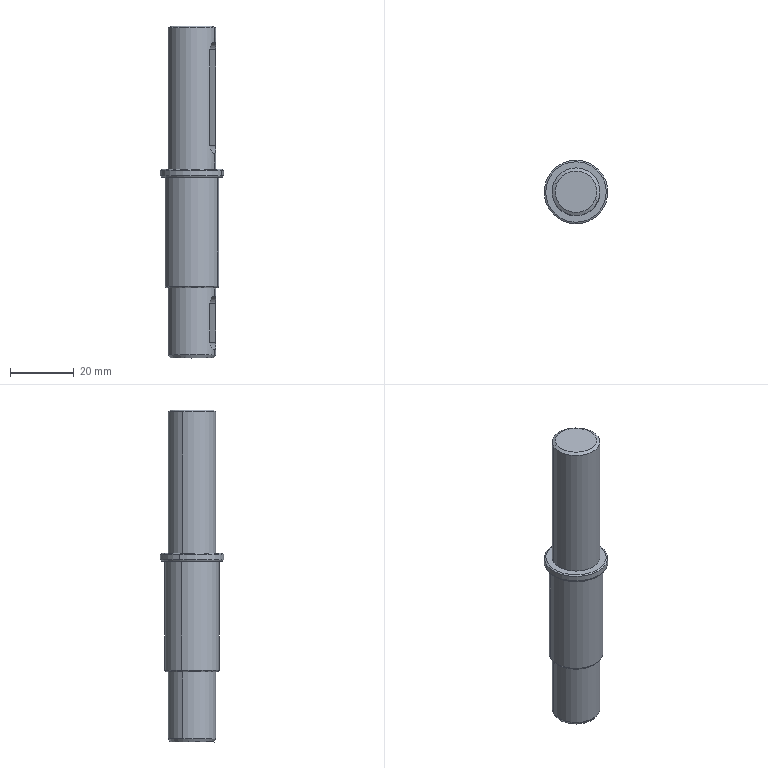Component | SolidWorks | 170423A4-ConveyorSynchronousPulleyAssembly-1_170423A4-PulleyFixedAxis1-1 | 1 solid | 35 faces | box 20 x 20 x 104.2 mm | volume 19748 mm3 | cylinder 14 | plane 11 | cone 10 | commonest cylinder face diameters 5 x6 15 x4 17 x2 20 x2
build123d program:
from build123d import *
from OCP.BRepFilletAPI import BRepFilletAPI_MakeChamfer

# Parameters (mm, degrees)
SKETCH1_R           = 7.5
BOSS_EXTRUDE1_DEPTH = 45
SKETCH2_R           = 10
BOSS_EXTRUDE2_DEPTH = 2.5
SKETCH3_R           = 8.5
BOSS_EXTRUDE3_DEPTH = 34.7
SKETCH4_R           = 7.5
BOSS_EXTRUDE4_DEPTH = 22
CHAMFER1_SIZE       = 1
CHAMFER1_SIZE2      = 0.5774
CHAMFER2_SIZE       = 0.5
CHAMFER2_SIZE2      = 0.2887
CUT_EXTRUDE3_DEPTH  = 3


with BuildPart() as part:
    # Sketch1 → Boss-Extrude1 (new body)
    with BuildSketch(Plane.XY):
        with Locations(Location((0, 0, 0), (0, 0, 180))):
            Circle(SKETCH1_R)
    extrude(amount=BOSS_EXTRUDE1_DEPTH)

    # Sketch2 → Boss-Extrude2 (add)
    with BuildSketch(Plane.XY.offset(45)):
        Circle(SKETCH2_R)
    extrude(amount=BOSS_EXTRUDE2_DEPTH)

    # Sketch3 → Boss-Extrude3 (add)
    with BuildSketch(Plane.XY.offset(47.5)):
        Circle(SKETCH3_R)
    extrude(amount=BOSS_EXTRUDE3_DEPTH)

    # Sketch4 → Boss-Extrude4 (add)
    with BuildSketch(Plane.XY.offset(82.2)):
        with Locations(Location((0, 0, 0), (0, 0, 180))):
            Circle(SKETCH4_R)
    extrude(amount=BOSS_EXTRUDE4_DEPTH)

    # Chamfer1: one chamfer whose edges measure the first distance from different faces: ONE call of the kernel's chamfer builder (chamfer() names one face for all edges)
    chamfer1_edges_1 = [part.edges().sort_by_distance(p)[0] for p in [
        (7.5, 0, 104.2),
    ]]
    chamfer1_side_1 = [part.faces().sort_by_distance(p)[0] for p in [
        (7.5, 0, 93.2),
    ]]
    chamfer1_edges_2 = [part.edges().sort_by_distance(p)[0] for p in [
        (7.5, 0, 0),
    ]]
    chamfer1_side_2 = [part.faces().sort_by_distance(p)[0] for p in [
        (0, 0, 0),
    ]]
    chamfer1 = BRepFilletAPI_MakeChamfer(part.part.solid().wrapped)
    for e in chamfer1_edges_1:
        chamfer1.Add(CHAMFER1_SIZE, CHAMFER1_SIZE2, e.wrapped, chamfer1_side_1[0].wrapped)  # the first distance lies on this face
    for e in chamfer1_edges_2:
        chamfer1.Add(CHAMFER1_SIZE, CHAMFER1_SIZE2, e.wrapped, chamfer1_side_2[0].wrapped)  # the first distance lies on this face
    add(Compound.cast(chamfer1.Shape()), mode=Mode.REPLACE)

    # Chamfer2: one chamfer whose edges measure the first distance from different faces: ONE call of the kernel's chamfer builder (chamfer() names one face for all edges)
    chamfer2_edges_1 = [part.edges().sort_by_distance(p)[0] for p in [
        (-8.5, 0, 82.2),
    ]]
    chamfer2_side_1 = [part.faces().sort_by_distance(p)[0] for p in [
        (-8.5, 0, 64.85),
    ]]
    chamfer2_edges_2 = [part.edges().sort_by_distance(p)[0] for p in [
        (-10, 0, 45),
    ]]
    chamfer2_side_2 = [part.faces().sort_by_distance(p)[0] for p in [
        (-9.717, 0, 45),
    ]]
    chamfer2_edges_3 = [part.edges().sort_by_distance(p)[0] for p in [
        (-10, 0, 47.5),
    ]]
    chamfer2_side_3 = [part.faces().sort_by_distance(p)[0] for p in [
        (-10, 0, 46.25),
    ]]
    chamfer2 = BRepFilletAPI_MakeChamfer(part.part.solid().wrapped)
    for e in chamfer2_edges_1:
        chamfer2.Add(CHAMFER2_SIZE, CHAMFER2_SIZE2, e.wrapped, chamfer2_side_1[0].wrapped)  # the first distance lies on this face
    for e in chamfer2_edges_2:
        chamfer2.Add(CHAMFER2_SIZE, CHAMFER2_SIZE2, e.wrapped, chamfer2_side_2[0].wrapped)  # the first distance lies on this face
    for e in chamfer2_edges_3:
        chamfer2.Add(CHAMFER2_SIZE, CHAMFER2_SIZE2, e.wrapped, chamfer2_side_3[0].wrapped)  # the first distance lies on this face
    add(Compound.cast(chamfer2.Shape()), mode=Mode.REPLACE)

    # Sketch8 → Cut-Extrude3 (cut)
    with BuildSketch(Plane(origin=(-7.5, 0, 0), x_dir=(0, 0, -1), z_dir=(1, 0, 0))):
        with BuildLine():
            Line((-99.2, 2.5), (-87.2, 2.5))
            ThreePointArc((-87.2, 2.5), (-84.7, 0), (-87.2, -2.5))
            Line((-87.2, -2.5), (-99.2, -2.5))
            ThreePointArc((-99.2, -2.5), (-101.7, 0), (-99.2, 2.5))
        make_face()
        with BuildLine():
            Line((-37.5, 2.5), (-7.5, 2.5))
            ThreePointArc((-7.5, 2.5), (-5, 0), (-7.5, -2.5))
            Line((-7.5, -2.5), (-37.5, -2.5))
            ThreePointArc((-37.5, -2.5), (-40, 0), (-37.5, 2.5))
        make_face()
    extrude(amount=CUT_EXTRUDE3_DEPTH, mode=Mode.SUBTRACT)


solid = part.part

# Placed as in the assembly
solid = solid.moved(Location((99.754, -120.788, 466.5), (-180, 0, -157.477)))